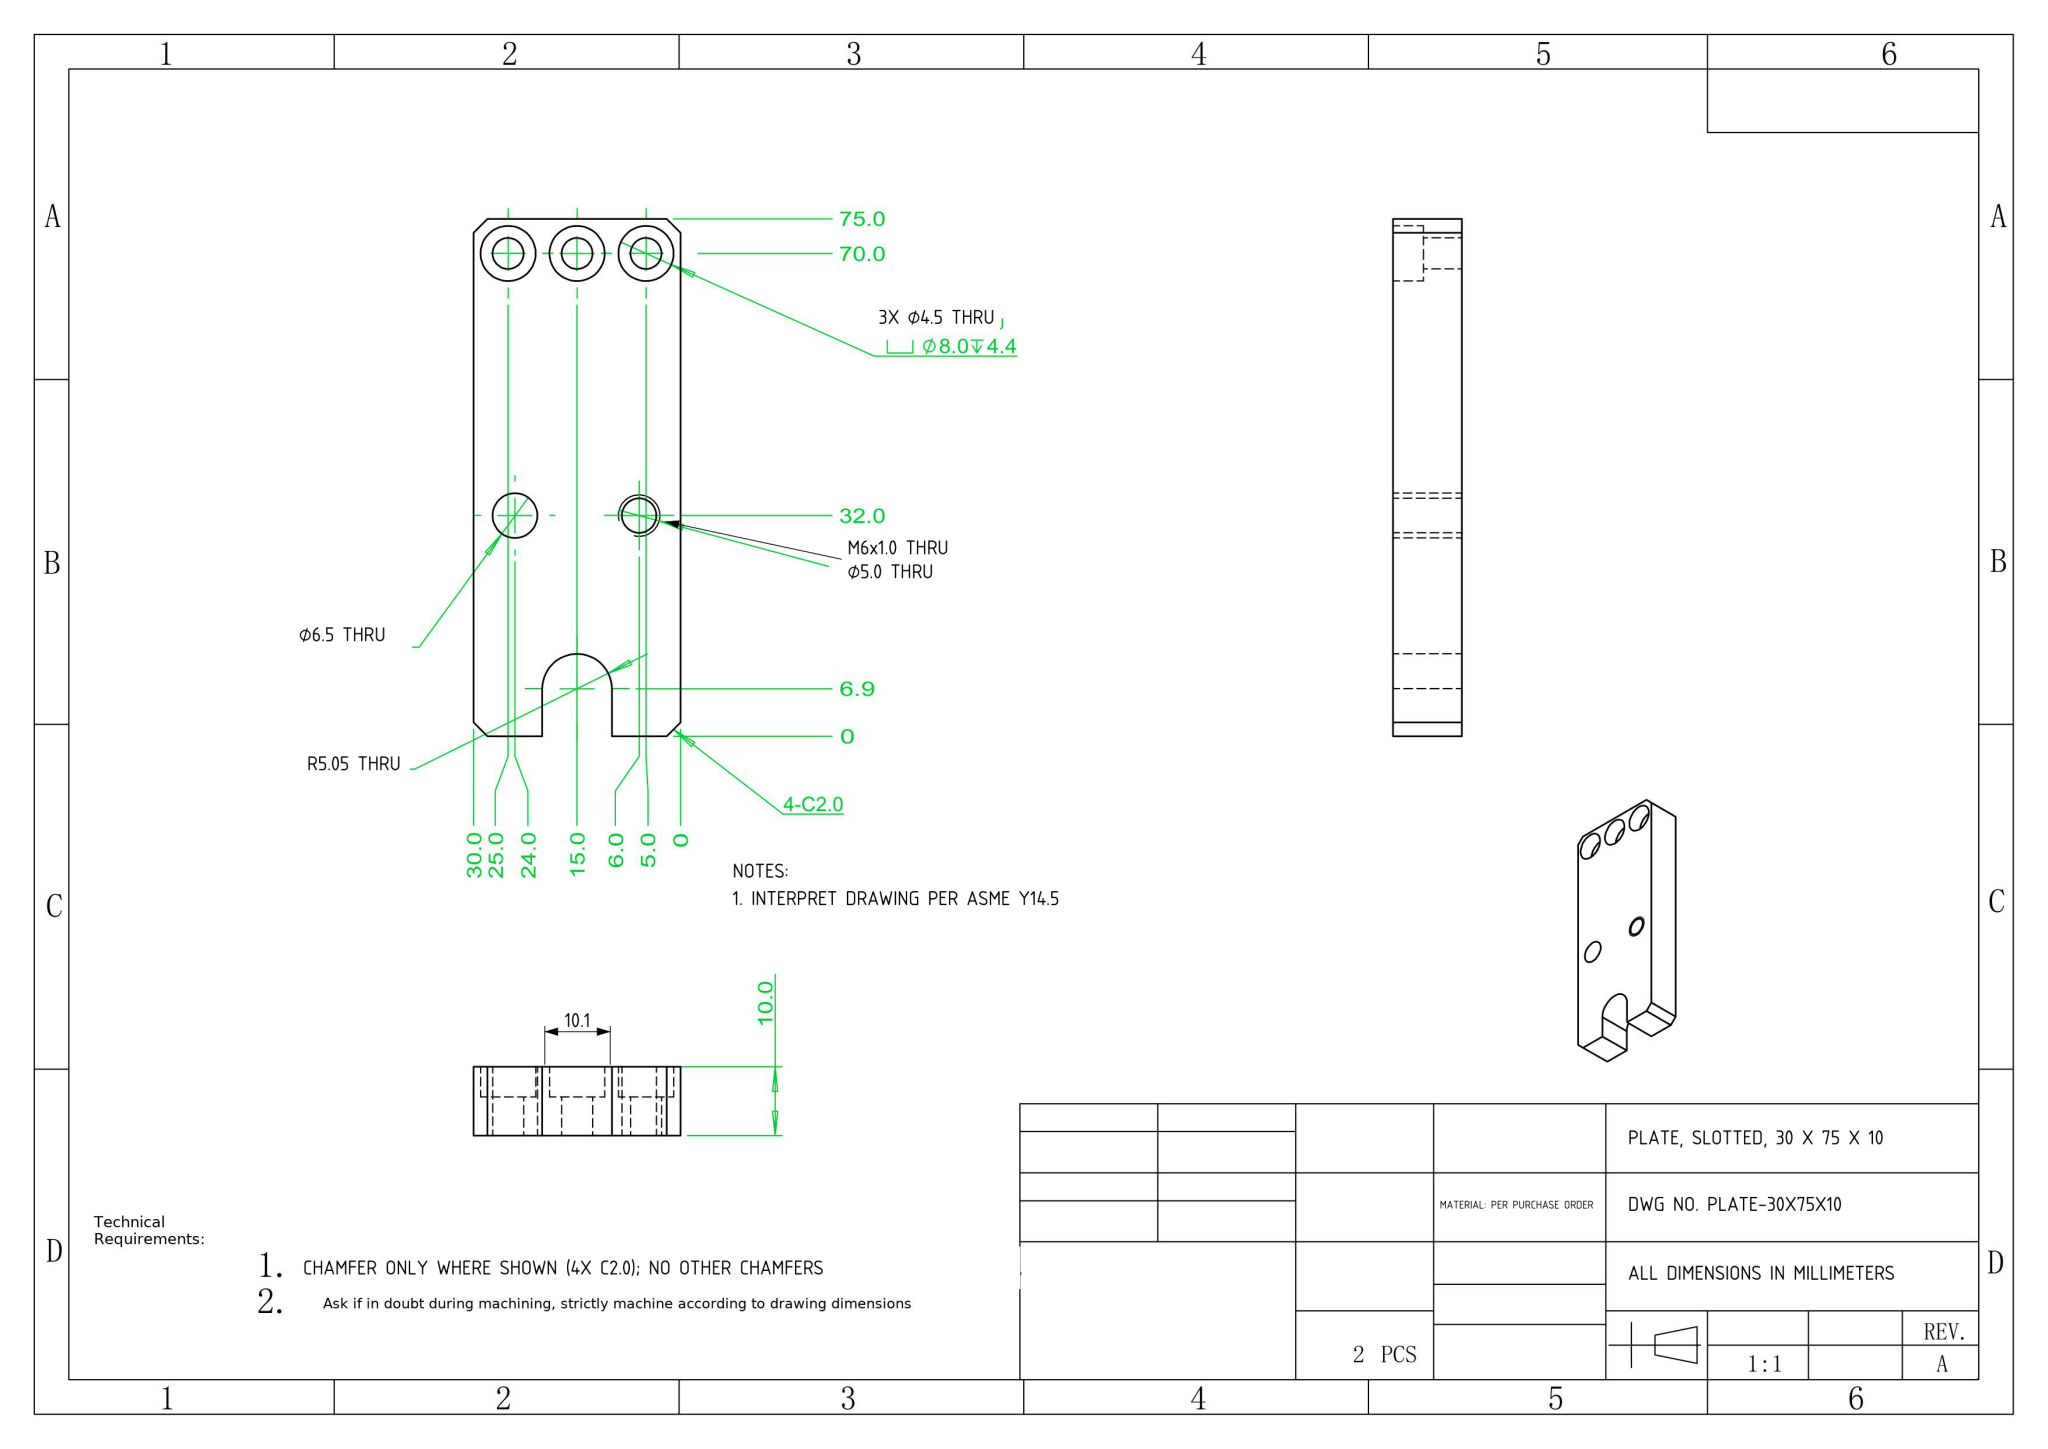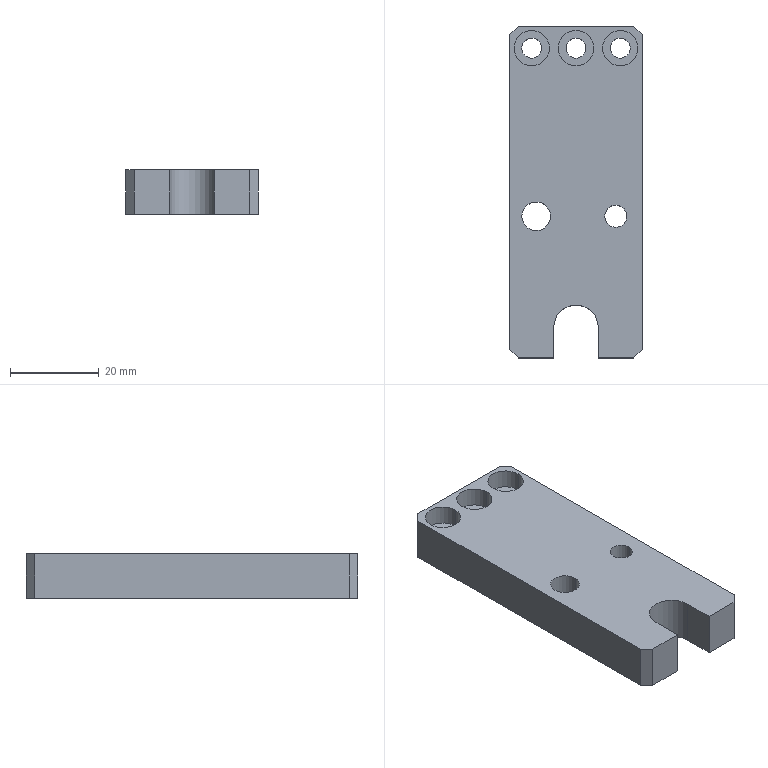Part | NX | mm | 1 solid | 33 faces | box 30 x 75 x 10 mm | volume 19864 mm3 | cylinder 17 | plane 16 | commonest cylinder face diameters 4.5 x6 8 x6 6.5 x2 5 x2 10.1 x1